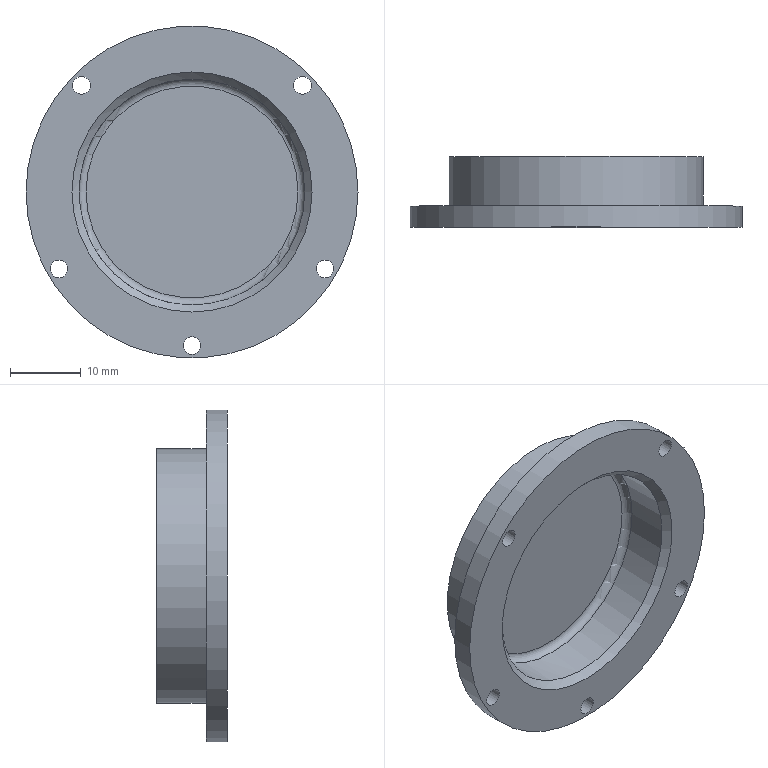Component | NX | FLANGE | 1 solid | 14 faces | box 47 x 10 x 47 mm | volume 5792 mm3 | cylinder 8 | plane 4 | cone 1 | torus 1 | commonest cylinder face diameters 2.5 x5 36 x1 47 x1 32 x1
STEP:
#1=CARTESIAN_POINT('',(0.,0.,0.));
#2=DIRECTION('',(0.,0.,1.));
#3=DIRECTION('',(1.,0.,0.));
#4=AXIS2_PLACEMENT_3D('',#1,#2,#3);
#5=CARTESIAN_POINT('',(-14.395,-16.2,58.409));
#6=VERTEX_POINT('',#5);
#7=CARTESIAN_POINT('',(-15.645,-16.2,58.409));
#8=DIRECTION('',(0.,1.,0.));
#9=DIRECTION('',(1.,0.,0.));
#10=AXIS2_PLACEMENT_3D('',#7,#8,#9);
#11=CIRCLE('',#10,1.25);
#12=CARTESIAN_POINT('',(0.0005589,-16.2,43.3));
#13=DIRECTION('',(0.,-1.,0.));
#14=DIRECTION('',(1.,0.,0.));
#15=AXIS2_PLACEMENT_3D('',#12,#13,#14);
#16=PLANE('',#15);
#17=CARTESIAN_POINT('',(-14.396,15.109));
#18=CARTESIAN_POINT('',(-14.396,12.944));
#19=CARTESIAN_POINT('',(-16.271,14.026));
#20=CARTESIAN_POINT('',(-18.146,15.109));
#21=CARTESIAN_POINT('',(-16.271,16.191));
#22=CARTESIAN_POINT('',(-14.396,17.274));
#23=CARTESIAN_POINT('',(-14.396,15.109));
#24=(BOUNDED_CURVE()B_SPLINE_CURVE(2,(#17,#18,#19,#20,#21,#22,#23),.UNSPECIFIED.,.T.,.F.)B_SPLINE_CURVE_WITH_KNOTS((1,2,2,2,2,1),(-2.094,0.,2.094,4.189,6.283,8.378),.UNSPECIFIED.)CURVE()GEOMETRIC_REPRESENTATION_ITEM()RATIONAL_B_SPLINE_CURVE((1.,0.5,1.,0.5,1.,0.5,1.))REPRESENTATION_ITEM(''));
#25=(GEOMETRIC_REPRESENTATION_CONTEXT(2)PARAMETRIC_REPRESENTATION_CONTEXT()REPRESENTATION_CONTEXT('',''));
#26=DEFINITIONAL_REPRESENTATION('',(#24),#25);
#27=PCURVE('',#16,#26);
#28=CARTESIAN_POINT('',(-15.645,-8.2,58.409));
#29=DIRECTION('',(0.,-1.,0.));
#30=DIRECTION('',(1.,0.,0.));
#31=AXIS2_PLACEMENT_3D('',#28,#29,#30);
#32=CYLINDRICAL_SURFACE('',#31,1.25);
#33=CARTESIAN_POINT('',(6.283,8.));
#34=DIRECTION('',(-1.,0.));
#35=VECTOR('',#34,1.);
#36=LINE('',#33,#35);
#37=(GEOMETRIC_REPRESENTATION_CONTEXT(2)PARAMETRIC_REPRESENTATION_CONTEXT()REPRESENTATION_CONTEXT('',''));
#38=DEFINITIONAL_REPRESENTATION('',(#36),#37);
#39=PCURVE('',#32,#38);
#40=SURFACE_CURVE('',#11,(#27,#39),.PCURVE_S1.);
#41=EDGE_CURVE('',#6,#6,#40,.T.);
#42=ORIENTED_EDGE('',*,*,#41,.T.);
#43=EDGE_LOOP('',(#42));
#44=FACE_BOUND('',#43,.T.);
#45=CARTESIAN_POINT('',(-17.585,-16.2,32.425));
#46=VERTEX_POINT('',#45);
#47=CARTESIAN_POINT('',(-18.835,-16.2,32.425));
#48=DIRECTION('',(0.,1.,0.));
#49=DIRECTION('',(1.,0.,0.));
#50=AXIS2_PLACEMENT_3D('',#47,#48,#49);
#51=CIRCLE('',#50,1.25);
#52=CARTESIAN_POINT('',(-17.586,-10.875));
#53=CARTESIAN_POINT('',(-17.586,-13.04));
#54=CARTESIAN_POINT('',(-19.461,-11.958));
#55=CARTESIAN_POINT('',(-21.336,-10.875));
#56=CARTESIAN_POINT('',(-19.461,-9.792));
#57=CARTESIAN_POINT('',(-17.586,-8.71));
#58=CARTESIAN_POINT('',(-17.586,-10.875));
#59=(BOUNDED_CURVE()B_SPLINE_CURVE(2,(#52,#53,#54,#55,#56,#57,#58),.UNSPECIFIED.,.T.,.F.)B_SPLINE_CURVE_WITH_KNOTS((1,2,2,2,2,1),(-2.094,0.,2.094,4.189,6.283,8.378),.UNSPECIFIED.)CURVE()GEOMETRIC_REPRESENTATION_ITEM()RATIONAL_B_SPLINE_CURVE((1.,0.5,1.,0.5,1.,0.5,1.))REPRESENTATION_ITEM(''));
#60=(GEOMETRIC_REPRESENTATION_CONTEXT(2)PARAMETRIC_REPRESENTATION_CONTEXT()REPRESENTATION_CONTEXT('',''));
#61=DEFINITIONAL_REPRESENTATION('',(#59),#60);
#62=PCURVE('',#16,#61);
#63=CARTESIAN_POINT('',(-18.835,-8.2,32.425));
#64=DIRECTION('',(0.,-1.,0.));
#65=DIRECTION('',(1.,0.,0.));
#66=AXIS2_PLACEMENT_3D('',#63,#64,#65);
#67=CYLINDRICAL_SURFACE('',#66,1.25);
#68=CARTESIAN_POINT('',(6.283,8.));
#69=DIRECTION('',(-1.,0.));
#70=VECTOR('',#69,1.);
#71=LINE('',#68,#70);
#72=(GEOMETRIC_REPRESENTATION_CONTEXT(2)PARAMETRIC_REPRESENTATION_CONTEXT()REPRESENTATION_CONTEXT('',''));
#73=DEFINITIONAL_REPRESENTATION('',(#71),#72);
#74=PCURVE('',#67,#73);
#75=SURFACE_CURVE('',#51,(#62,#74),.PCURVE_S1.);
#76=EDGE_CURVE('',#46,#46,#75,.T.);
#77=ORIENTED_EDGE('',*,*,#76,.T.);
#78=EDGE_LOOP('',(#77));
#79=FACE_BOUND('',#78,.T.);
#80=CARTESIAN_POINT('',(1.251,-16.2,21.55));
#81=VERTEX_POINT('',#80);
#82=CARTESIAN_POINT('',(0.0005589,-16.2,21.55));
#83=DIRECTION('',(0.,1.,0.));
#84=DIRECTION('',(1.,0.,0.));
#85=AXIS2_PLACEMENT_3D('',#82,#83,#84);
#86=CIRCLE('',#85,1.25);
#87=CARTESIAN_POINT('',(1.25,-21.75));
#88=CARTESIAN_POINT('',(1.25,-23.915));
#89=CARTESIAN_POINT('',(-0.625,-22.833));
#90=CARTESIAN_POINT('',(-2.5,-21.75));
#91=CARTESIAN_POINT('',(-0.625,-20.667));
#92=CARTESIAN_POINT('',(1.25,-19.585));
#93=CARTESIAN_POINT('',(1.25,-21.75));
#94=(BOUNDED_CURVE()B_SPLINE_CURVE(2,(#87,#88,#89,#90,#91,#92,#93),.UNSPECIFIED.,.T.,.F.)B_SPLINE_CURVE_WITH_KNOTS((1,2,2,2,2,1),(-2.094,0.,2.094,4.189,6.283,8.378),.UNSPECIFIED.)CURVE()GEOMETRIC_REPRESENTATION_ITEM()RATIONAL_B_SPLINE_CURVE((1.,0.5,1.,0.5,1.,0.5,1.))REPRESENTATION_ITEM(''));
#95=(GEOMETRIC_REPRESENTATION_CONTEXT(2)PARAMETRIC_REPRESENTATION_CONTEXT()REPRESENTATION_CONTEXT('',''));
#96=DEFINITIONAL_REPRESENTATION('',(#94),#95);
#97=PCURVE('',#16,#96);
#98=CARTESIAN_POINT('',(0.0005589,-8.2,21.55));
#99=DIRECTION('',(0.,-1.,0.));
#100=DIRECTION('',(1.,0.,0.));
#101=AXIS2_PLACEMENT_3D('',#98,#99,#100);
#102=CYLINDRICAL_SURFACE('',#101,1.25);
#103=CARTESIAN_POINT('',(6.283,8.));
#104=DIRECTION('',(-1.,0.));
#105=VECTOR('',#104,1.);
#106=LINE('',#103,#105);
#107=(GEOMETRIC_REPRESENTATION_CONTEXT(2)PARAMETRIC_REPRESENTATION_CONTEXT()REPRESENTATION_CONTEXT('',''));
#108=DEFINITIONAL_REPRESENTATION('',(#106),#107);
#109=PCURVE('',#102,#108);
#110=SURFACE_CURVE('',#86,(#97,#109),.PCURVE_S1.);
#111=EDGE_CURVE('',#81,#81,#110,.T.);
#112=ORIENTED_EDGE('',*,*,#111,.T.);
#113=EDGE_LOOP('',(#112));
#114=FACE_BOUND('',#113,.T.);
#115=CARTESIAN_POINT('',(17.001,-16.2,43.3));
#116=VERTEX_POINT('',#115);
#117=CARTESIAN_POINT('',(0.0005589,-16.2,43.3));
#118=DIRECTION('',(0.,1.,0.));
#119=DIRECTION('',(1.,0.,0.));
#120=AXIS2_PLACEMENT_3D('',#117,#118,#119);
#121=CIRCLE('',#120,17.);
#122=CARTESIAN_POINT('',(17.,0.));
#123=CARTESIAN_POINT('',(17.,-29.445));
#124=CARTESIAN_POINT('',(-8.5,-14.722));
#125=CARTESIAN_POINT('',(-34.,-0.));
#126=CARTESIAN_POINT('',(-8.5,14.722));
#127=CARTESIAN_POINT('',(17.,29.445));
#128=CARTESIAN_POINT('',(17.,0.));
#129=(BOUNDED_CURVE()B_SPLINE_CURVE(2,(#122,#123,#124,#125,#126,#127,#128),.UNSPECIFIED.,.T.,.F.)B_SPLINE_CURVE_WITH_KNOTS((1,2,2,2,2,1),(-2.094,0.,2.094,4.189,6.283,8.378),.UNSPECIFIED.)CURVE()GEOMETRIC_REPRESENTATION_ITEM()RATIONAL_B_SPLINE_CURVE((1.,0.5,1.,0.5,1.,0.5,1.))REPRESENTATION_ITEM(''));
#130=(GEOMETRIC_REPRESENTATION_CONTEXT(2)PARAMETRIC_REPRESENTATION_CONTEXT()REPRESENTATION_CONTEXT('',''));
#131=DEFINITIONAL_REPRESENTATION('',(#129),#130);
#132=PCURVE('',#16,#131);
#133=CARTESIAN_POINT('',(0.0005589,-16.2,43.3));
#134=DIRECTION('',(0.,-1.,0.));
#135=DIRECTION('',(1.,0.,0.));
#136=AXIS2_PLACEMENT_3D('',#133,#134,#135);
#137=CONICAL_SURFACE('',#136,17.,0.7854);
#138=CARTESIAN_POINT('',(6.283,0.));
#139=DIRECTION('',(-1.,0.));
#140=VECTOR('',#139,1.);
#141=LINE('',#138,#140);
#142=(GEOMETRIC_REPRESENTATION_CONTEXT(2)PARAMETRIC_REPRESENTATION_CONTEXT()REPRESENTATION_CONTEXT('',''));
#143=DEFINITIONAL_REPRESENTATION('',(#141),#142);
#144=PCURVE('',#137,#143);
#145=SURFACE_CURVE('',#121,(#132,#144),.PCURVE_S1.);
#146=EDGE_CURVE('',#116,#116,#145,.T.);
#147=ORIENTED_EDGE('',*,*,#146,.T.);
#148=EDGE_LOOP('',(#147));
#149=FACE_BOUND('',#148,.T.);
#150=CARTESIAN_POINT('',(23.501,-16.2,43.3));
#151=VERTEX_POINT('',#150);
#152=CARTESIAN_POINT('',(0.0005589,-16.2,43.3));
#153=DIRECTION('',(0.,-1.,0.));
#154=DIRECTION('',(1.,0.,0.));
#155=AXIS2_PLACEMENT_3D('',#152,#153,#154);
#156=CIRCLE('',#155,23.5);
#157=CARTESIAN_POINT('',(0.,0.));
#158=DIRECTION('',(1.,0.));
#159=AXIS2_PLACEMENT_2D('',#157,#158);
#160=CIRCLE('',#159,23.5);
#161=(GEOMETRIC_REPRESENTATION_CONTEXT(2)PARAMETRIC_REPRESENTATION_CONTEXT()REPRESENTATION_CONTEXT('',''));
#162=DEFINITIONAL_REPRESENTATION('',(#160),#161);
#163=PCURVE('',#16,#162);
#164=CARTESIAN_POINT('',(0.0005589,-13.2,43.3));
#165=DIRECTION('',(0.,-1.,0.));
#166=DIRECTION('',(1.,0.,0.));
#167=AXIS2_PLACEMENT_3D('',#164,#165,#166);
#168=CYLINDRICAL_SURFACE('',#167,23.5);
#169=CARTESIAN_POINT('',(0.,3.));
#170=DIRECTION('',(1.,0.));
#171=VECTOR('',#170,1.);
#172=LINE('',#169,#171);
#173=(GEOMETRIC_REPRESENTATION_CONTEXT(2)PARAMETRIC_REPRESENTATION_CONTEXT()REPRESENTATION_CONTEXT('',''));
#174=DEFINITIONAL_REPRESENTATION('',(#172),#173);
#175=PCURVE('',#168,#174);
#176=SURFACE_CURVE('',#156,(#163,#175),.PCURVE_S1.);
#177=EDGE_CURVE('',#151,#151,#176,.T.);
#178=ORIENTED_EDGE('',*,*,#177,.T.);
#179=EDGE_LOOP('',(#178));
#180=FACE_BOUND('',#179,.T.);
#181=CARTESIAN_POINT('',(14.396,-16.2,58.409));
#182=VERTEX_POINT('',#181);
#183=CARTESIAN_POINT('',(15.646,-16.2,58.409));
#184=DIRECTION('',(0.,-1.,0.));
#185=DIRECTION('',(-1.,0.,0.));
#186=AXIS2_PLACEMENT_3D('',#183,#184,#185);
#187=CIRCLE('',#186,1.25);
#188=CARTESIAN_POINT('',(15.646,15.109));
#189=DIRECTION('',(-1.,0.));
#190=AXIS2_PLACEMENT_2D('',#188,#189);
#191=CIRCLE('',#190,1.25);
#192=(GEOMETRIC_REPRESENTATION_CONTEXT(2)PARAMETRIC_REPRESENTATION_CONTEXT()REPRESENTATION_CONTEXT('',''));
#193=DEFINITIONAL_REPRESENTATION('',(#191),#192);
#194=PCURVE('',#16,#193);
#195=CARTESIAN_POINT('',(15.646,-8.2,58.409));
#196=DIRECTION('',(0.,-1.,0.));
#197=DIRECTION('',(1.,0.,0.));
#198=AXIS2_PLACEMENT_3D('',#195,#196,#197);
#199=CYLINDRICAL_SURFACE('',#198,1.25);
#200=CARTESIAN_POINT('',(3.142,8.));
#201=DIRECTION('',(1.,0.));
#202=VECTOR('',#201,1.);
#203=LINE('',#200,#202);
#204=(GEOMETRIC_REPRESENTATION_CONTEXT(2)PARAMETRIC_REPRESENTATION_CONTEXT()REPRESENTATION_CONTEXT('',''));
#205=DEFINITIONAL_REPRESENTATION('',(#203),#204);
#206=PCURVE('',#199,#205);
#207=SURFACE_CURVE('',#187,(#194,#206),.PCURVE_S1.);
#208=EDGE_CURVE('',#182,#182,#207,.T.);
#209=ORIENTED_EDGE('',*,*,#208,.F.);
#210=EDGE_LOOP('',(#209));
#211=FACE_BOUND('',#210,.T.);
#212=CARTESIAN_POINT('',(17.587,-16.2,32.425));
#213=VERTEX_POINT('',#212);
#214=CARTESIAN_POINT('',(18.837,-16.2,32.425));
#215=DIRECTION('',(0.,-1.,0.));
#216=DIRECTION('',(-1.,0.,0.));
#217=AXIS2_PLACEMENT_3D('',#214,#215,#216);
#218=CIRCLE('',#217,1.25);
#219=CARTESIAN_POINT('',(18.836,-10.875));
#220=DIRECTION('',(-1.,0.));
#221=AXIS2_PLACEMENT_2D('',#219,#220);
#222=CIRCLE('',#221,1.25);
#223=(GEOMETRIC_REPRESENTATION_CONTEXT(2)PARAMETRIC_REPRESENTATION_CONTEXT()REPRESENTATION_CONTEXT('',''));
#224=DEFINITIONAL_REPRESENTATION('',(#222),#223);
#225=PCURVE('',#16,#224);
#226=CARTESIAN_POINT('',(18.837,-8.2,32.425));
#227=DIRECTION('',(0.,-1.,0.));
#228=DIRECTION('',(1.,0.,0.));
#229=AXIS2_PLACEMENT_3D('',#226,#227,#228);
#230=CYLINDRICAL_SURFACE('',#229,1.25);
#231=CARTESIAN_POINT('',(3.142,8.));
#232=DIRECTION('',(1.,0.));
#233=VECTOR('',#232,1.);
#234=LINE('',#231,#233);
#235=(GEOMETRIC_REPRESENTATION_CONTEXT(2)PARAMETRIC_REPRESENTATION_CONTEXT()REPRESENTATION_CONTEXT('',''));
#236=DEFINITIONAL_REPRESENTATION('',(#234),#235);
#237=PCURVE('',#230,#236);
#238=SURFACE_CURVE('',#218,(#225,#237),.PCURVE_S1.);
#239=EDGE_CURVE('',#213,#213,#238,.T.);
#240=ORIENTED_EDGE('',*,*,#239,.F.);
#241=EDGE_LOOP('',(#240));
#242=FACE_BOUND('',#241,.T.);
#243=ADVANCED_FACE('',(#44,#79,#114,#149,#180,#211,#242),#16,.T.);
#244=CARTESIAN_POINT('',(-16.895,-13.2,58.409));
#245=VERTEX_POINT('',#244);
#246=CARTESIAN_POINT('',(-14.395,-13.2,58.409));
#247=VERTEX_POINT('',#246);
#248=CARTESIAN_POINT('',(-15.645,-13.2,58.409));
#249=DIRECTION('',(0.,-1.,0.));
#250=DIRECTION('',(-1.,0.,0.));
#251=AXIS2_PLACEMENT_3D('',#248,#249,#250);
#252=CIRCLE('',#251,1.25);
#253=CARTESIAN_POINT('',(0.0005589,-13.2,43.3));
#254=DIRECTION('',(0.,1.,0.));
#255=DIRECTION('',(-1.,0.,0.));
#256=AXIS2_PLACEMENT_3D('',#253,#254,#255);
#257=PLANE('',#256);
#258=CARTESIAN_POINT('',(16.896,15.109));
#259=CARTESIAN_POINT('',(16.896,12.944));
#260=CARTESIAN_POINT('',(15.021,14.026));
#261=CARTESIAN_POINT('',(13.146,15.109));
#262=CARTESIAN_POINT('',(15.021,16.191));
#263=CARTESIAN_POINT('',(16.896,17.274));
#264=CARTESIAN_POINT('',(16.896,15.109));
#265=(BOUNDED_CURVE()B_SPLINE_CURVE(2,(#258,#259,#260,#261,#262,#263,#264),.UNSPECIFIED.,.T.,.F.)B_SPLINE_CURVE_WITH_KNOTS((1,2,2,2,2,1),(-2.094,0.,2.094,4.189,6.283,8.378),.UNSPECIFIED.)CURVE()GEOMETRIC_REPRESENTATION_ITEM()RATIONAL_B_SPLINE_CURVE((1.,0.5,1.,0.5,1.,0.5,1.))REPRESENTATION_ITEM(''));
#266=(GEOMETRIC_REPRESENTATION_CONTEXT(2)PARAMETRIC_REPRESENTATION_CONTEXT()REPRESENTATION_CONTEXT('',''));
#267=DEFINITIONAL_REPRESENTATION('',(#265),#266);
#268=PCURVE('',#257,#267);
#269=CARTESIAN_POINT('',(3.142,5.));
#270=DIRECTION('',(1.,0.));
#271=VECTOR('',#270,1.);
#272=LINE('',#269,#271);
#273=(GEOMETRIC_REPRESENTATION_CONTEXT(2)PARAMETRIC_REPRESENTATION_CONTEXT()REPRESENTATION_CONTEXT('',''));
#274=DEFINITIONAL_REPRESENTATION('',(#272),#273);
#275=PCURVE('',#32,#274);
#276=SURFACE_CURVE('',#252,(#268,#275),.PCURVE_S1.);
#277=EDGE_CURVE('',#245,#247,#276,.T.);
#278=ORIENTED_EDGE('',*,*,#277,.T.);
#279=CARTESIAN_POINT('',(-15.645,-13.2,58.409));
#280=DIRECTION('',(0.,-1.,0.));
#281=DIRECTION('',(-1.,0.,0.));
#282=AXIS2_PLACEMENT_3D('',#279,#280,#281);
#283=CIRCLE('',#282,1.25);
#284=CARTESIAN_POINT('',(16.896,15.109));
#285=CARTESIAN_POINT('',(16.896,12.944));
#286=CARTESIAN_POINT('',(15.021,14.026));
#287=CARTESIAN_POINT('',(13.146,15.109));
#288=CARTESIAN_POINT('',(15.021,16.191));
#289=CARTESIAN_POINT('',(16.896,17.274));
#290=CARTESIAN_POINT('',(16.896,15.109));
#291=(BOUNDED_CURVE()B_SPLINE_CURVE(2,(#284,#285,#286,#287,#288,#289,#290),.UNSPECIFIED.,.T.,.F.)B_SPLINE_CURVE_WITH_KNOTS((1,2,2,2,2,1),(-2.094,0.,2.094,4.189,6.283,8.378),.UNSPECIFIED.)CURVE()GEOMETRIC_REPRESENTATION_ITEM()RATIONAL_B_SPLINE_CURVE((1.,0.5,1.,0.5,1.,0.5,1.))REPRESENTATION_ITEM(''));
#292=(GEOMETRIC_REPRESENTATION_CONTEXT(2)PARAMETRIC_REPRESENTATION_CONTEXT()REPRESENTATION_CONTEXT('',''));
#293=DEFINITIONAL_REPRESENTATION('',(#291),#292);
#294=PCURVE('',#257,#293);
#295=CARTESIAN_POINT('',(-3.142,5.));
#296=DIRECTION('',(1.,0.));
#297=VECTOR('',#296,1.);
#298=LINE('',#295,#297);
#299=(GEOMETRIC_REPRESENTATION_CONTEXT(2)PARAMETRIC_REPRESENTATION_CONTEXT()REPRESENTATION_CONTEXT('',''));
#300=DEFINITIONAL_REPRESENTATION('',(#298),#299);
#301=PCURVE('',#32,#300);
#302=SURFACE_CURVE('',#283,(#294,#301),.PCURVE_S1.);
#303=EDGE_CURVE('',#247,#245,#302,.T.);
#304=ORIENTED_EDGE('',*,*,#303,.T.);
#305=EDGE_LOOP('',(#278,#304));
#306=FACE_BOUND('',#305,.T.);
#307=CARTESIAN_POINT('',(-20.085,-13.2,32.425));
#308=VERTEX_POINT('',#307);
#309=CARTESIAN_POINT('',(-17.585,-13.2,32.425));
#310=VERTEX_POINT('',#309);
#311=CARTESIAN_POINT('',(-18.835,-13.2,32.425));
#312=DIRECTION('',(0.,-1.,0.));
#313=DIRECTION('',(-1.,0.,0.));
#314=AXIS2_PLACEMENT_3D('',#311,#312,#313);
#315=CIRCLE('',#314,1.25);
#316=CARTESIAN_POINT('',(20.086,-10.875));
#317=CARTESIAN_POINT('',(20.086,-13.04));
#318=CARTESIAN_POINT('',(18.211,-11.958));
#319=CARTESIAN_POINT('',(16.336,-10.875));
#320=CARTESIAN_POINT('',(18.211,-9.792));
#321=CARTESIAN_POINT('',(20.086,-8.71));
#322=CARTESIAN_POINT('',(20.086,-10.875));
#323=(BOUNDED_CURVE()B_SPLINE_CURVE(2,(#316,#317,#318,#319,#320,#321,#322),.UNSPECIFIED.,.T.,.F.)B_SPLINE_CURVE_WITH_KNOTS((1,2,2,2,2,1),(-2.094,0.,2.094,4.189,6.283,8.378),.UNSPECIFIED.)CURVE()GEOMETRIC_REPRESENTATION_ITEM()RATIONAL_B_SPLINE_CURVE((1.,0.5,1.,0.5,1.,0.5,1.))REPRESENTATION_ITEM(''));
#324=(GEOMETRIC_REPRESENTATION_CONTEXT(2)PARAMETRIC_REPRESENTATION_CONTEXT()REPRESENTATION_CONTEXT('',''));
#325=DEFINITIONAL_REPRESENTATION('',(#323),#324);
#326=PCURVE('',#257,#325);
#327=CARTESIAN_POINT('',(3.142,5.));
#328=DIRECTION('',(1.,0.));
#329=VECTOR('',#328,1.);
#330=LINE('',#327,#329);
#331=(GEOMETRIC_REPRESENTATION_CONTEXT(2)PARAMETRIC_REPRESENTATION_CONTEXT()REPRESENTATION_CONTEXT('',''));
#332=DEFINITIONAL_REPRESENTATION('',(#330),#331);
#333=PCURVE('',#67,#332);
#334=SURFACE_CURVE('',#315,(#326,#333),.PCURVE_S1.);
#335=EDGE_CURVE('',#308,#310,#334,.T.);
#336=ORIENTED_EDGE('',*,*,#335,.T.);
#337=CARTESIAN_POINT('',(-18.835,-13.2,32.425));
#338=DIRECTION('',(0.,-1.,0.));
#339=DIRECTION('',(-1.,0.,0.));
#340=AXIS2_PLACEMENT_3D('',#337,#338,#339);
#341=CIRCLE('',#340,1.25);
#342=CARTESIAN_POINT('',(20.086,-10.875));
#343=CARTESIAN_POINT('',(20.086,-13.04));
#344=CARTESIAN_POINT('',(18.211,-11.958));
#345=CARTESIAN_POINT('',(16.336,-10.875));
#346=CARTESIAN_POINT('',(18.211,-9.792));
#347=CARTESIAN_POINT('',(20.086,-8.71));
#348=CARTESIAN_POINT('',(20.086,-10.875));
#349=(BOUNDED_CURVE()B_SPLINE_CURVE(2,(#342,#343,#344,#345,#346,#347,#348),.UNSPECIFIED.,.T.,.F.)B_SPLINE_CURVE_WITH_KNOTS((1,2,2,2,2,1),(-2.094,0.,2.094,4.189,6.283,8.378),.UNSPECIFIED.)CURVE()GEOMETRIC_REPRESENTATION_ITEM()RATIONAL_B_SPLINE_CURVE((1.,0.5,1.,0.5,1.,0.5,1.))REPRESENTATION_ITEM(''));
#350=(GEOMETRIC_REPRESENTATION_CONTEXT(2)PARAMETRIC_REPRESENTATION_CONTEXT()REPRESENTATION_CONTEXT('',''));
#351=DEFINITIONAL_REPRESENTATION('',(#349),#350);
#352=PCURVE('',#257,#351);
#353=CARTESIAN_POINT('',(-3.142,5.));
#354=DIRECTION('',(1.,0.));
#355=VECTOR('',#354,1.);
#356=LINE('',#353,#355);
#357=(GEOMETRIC_REPRESENTATION_CONTEXT(2)PARAMETRIC_REPRESENTATION_CONTEXT()REPRESENTATION_CONTEXT('',''));
#358=DEFINITIONAL_REPRESENTATION('',(#356),#357);
#359=PCURVE('',#67,#358);
#360=SURFACE_CURVE('',#341,(#352,#359),.PCURVE_S1.);
#361=EDGE_CURVE('',#310,#308,#360,.T.);
#362=ORIENTED_EDGE('',*,*,#361,.T.);
#363=EDGE_LOOP('',(#336,#362));
#364=FACE_BOUND('',#363,.T.);
#365=CARTESIAN_POINT('',(-1.249,-13.2,21.55));
#366=VERTEX_POINT('',#365);
#367=CARTESIAN_POINT('',(1.251,-13.2,21.55));
#368=VERTEX_POINT('',#367);
#369=CARTESIAN_POINT('',(0.0005589,-13.2,21.55));
#370=DIRECTION('',(0.,-1.,0.));
#371=DIRECTION('',(-1.,0.,0.));
#372=AXIS2_PLACEMENT_3D('',#369,#370,#371);
#373=CIRCLE('',#372,1.25);
#374=CARTESIAN_POINT('',(1.25,-21.75));
#375=CARTESIAN_POINT('',(1.25,-23.915));
#376=CARTESIAN_POINT('',(-0.625,-22.833));
#377=CARTESIAN_POINT('',(-2.5,-21.75));
#378=CARTESIAN_POINT('',(-0.625,-20.667));
#379=CARTESIAN_POINT('',(1.25,-19.585));
#380=CARTESIAN_POINT('',(1.25,-21.75));
#381=(BOUNDED_CURVE()B_SPLINE_CURVE(2,(#374,#375,#376,#377,#378,#379,#380),.UNSPECIFIED.,.T.,.F.)B_SPLINE_CURVE_WITH_KNOTS((1,2,2,2,2,1),(-2.094,0.,2.094,4.189,6.283,8.378),.UNSPECIFIED.)CURVE()GEOMETRIC_REPRESENTATION_ITEM()RATIONAL_B_SPLINE_CURVE((1.,0.5,1.,0.5,1.,0.5,1.))REPRESENTATION_ITEM(''));
#382=(GEOMETRIC_REPRESENTATION_CONTEXT(2)PARAMETRIC_REPRESENTATION_CONTEXT()REPRESENTATION_CONTEXT('',''));
#383=DEFINITIONAL_REPRESENTATION('',(#381),#382);
#384=PCURVE('',#257,#383);
#385=CARTESIAN_POINT('',(3.142,5.));
#386=DIRECTION('',(1.,0.));
#387=VECTOR('',#386,1.);
#388=LINE('',#385,#387);
#389=(GEOMETRIC_REPRESENTATION_CONTEXT(2)PARAMETRIC_REPRESENTATION_CONTEXT()REPRESENTATION_CONTEXT('',''));
#390=DEFINITIONAL_REPRESENTATION('',(#388),#389);
#391=PCURVE('',#102,#390);
#392=SURFACE_CURVE('',#373,(#384,#391),.PCURVE_S1.);
#393=EDGE_CURVE('',#366,#368,#392,.T.);
#394=ORIENTED_EDGE('',*,*,#393,.T.);
#395=CARTESIAN_POINT('',(0.0005589,-13.2,21.55));
#396=DIRECTION('',(0.,-1.,0.));
#397=DIRECTION('',(-1.,0.,0.));
#398=AXIS2_PLACEMENT_3D('',#395,#396,#397);
#399=CIRCLE('',#398,1.25);
#400=CARTESIAN_POINT('',(1.25,-21.75));
#401=CARTESIAN_POINT('',(1.25,-23.915));
#402=CARTESIAN_POINT('',(-0.625,-22.833));
#403=CARTESIAN_POINT('',(-2.5,-21.75));
#404=CARTESIAN_POINT('',(-0.625,-20.667));
#405=CARTESIAN_POINT('',(1.25,-19.585));
#406=CARTESIAN_POINT('',(1.25,-21.75));
#407=(BOUNDED_CURVE()B_SPLINE_CURVE(2,(#400,#401,#402,#403,#404,#405,#406),.UNSPECIFIED.,.T.,.F.)B_SPLINE_CURVE_WITH_KNOTS((1,2,2,2,2,1),(-2.094,0.,2.094,4.189,6.283,8.378),.UNSPECIFIED.)CURVE()GEOMETRIC_REPRESENTATION_ITEM()RATIONAL_B_SPLINE_CURVE((1.,0.5,1.,0.5,1.,0.5,1.))REPRESENTATION_ITEM(''));
#408=(GEOMETRIC_REPRESENTATION_CONTEXT(2)PARAMETRIC_REPRESENTATION_CONTEXT()REPRESENTATION_CONTEXT('',''));
#409=DEFINITIONAL_REPRESENTATION('',(#407),#408);
#410=PCURVE('',#257,#409);
#411=CARTESIAN_POINT('',(-3.142,5.));
#412=DIRECTION('',(1.,0.));
#413=VECTOR('',#412,1.);
#414=LINE('',#411,#413);
#415=(GEOMETRIC_REPRESENTATION_CONTEXT(2)PARAMETRIC_REPRESENTATION_CONTEXT()REPRESENTATION_CONTEXT('',''));
#416=DEFINITIONAL_REPRESENTATION('',(#414),#415);
#417=PCURVE('',#102,#416);
#418=SURFACE_CURVE('',#399,(#410,#417),.PCURVE_S1.);
#419=EDGE_CURVE('',#368,#366,#418,.T.);
#420=ORIENTED_EDGE('',*,*,#419,.T.);
#421=EDGE_LOOP('',(#394,#420));
#422=FACE_BOUND('',#421,.T.);
#423=CARTESIAN_POINT('',(18.001,-13.2,43.3));
#424=VERTEX_POINT('',#423);
#425=CARTESIAN_POINT('',(0.0005589,-13.2,43.3));
#426=DIRECTION('',(0.,1.,0.));
#427=DIRECTION('',(1.,0.,0.));
#428=AXIS2_PLACEMENT_3D('',#425,#426,#427);
#429=CIRCLE('',#428,18.);
#430=CARTESIAN_POINT('',(0.,0.));
#431=DIRECTION('',(-1.,0.));
#432=AXIS2_PLACEMENT_2D('',#430,#431);
#433=CIRCLE('',#432,18.);
#434=(GEOMETRIC_REPRESENTATION_CONTEXT(2)PARAMETRIC_REPRESENTATION_CONTEXT()REPRESENTATION_CONTEXT('',''));
#435=DEFINITIONAL_REPRESENTATION('',(#433),#434);
#436=PCURVE('',#257,#435);
#437=CARTESIAN_POINT('',(0.0005589,-6.2,43.3));
#438=DIRECTION('',(0.,-1.,0.));
#439=DIRECTION('',(1.,0.,0.));
#440=AXIS2_PLACEMENT_3D('',#437,#438,#439);
#441=CYLINDRICAL_SURFACE('',#440,18.);
#442=CARTESIAN_POINT('',(6.283,7.));
#443=DIRECTION('',(-1.,0.));
#444=VECTOR('',#443,1.);
#445=LINE('',#442,#444);
#446=(GEOMETRIC_REPRESENTATION_CONTEXT(2)PARAMETRIC_REPRESENTATION_CONTEXT()REPRESENTATION_CONTEXT('',''));
#447=DEFINITIONAL_REPRESENTATION('',(#445),#446);
#448=PCURVE('',#441,#447);
#449=SURFACE_CURVE('',#429,(#436,#448),.PCURVE_S1.);
#450=EDGE_CURVE('',#424,#424,#449,.T.);
#451=ORIENTED_EDGE('',*,*,#450,.F.);
#452=EDGE_LOOP('',(#451));
#453=FACE_BOUND('',#452,.T.);
#454=CARTESIAN_POINT('',(23.501,-13.2,43.3));
#455=VERTEX_POINT('',#454);
#456=CARTESIAN_POINT('',(0.0005589,-13.2,43.3));
#457=DIRECTION('',(0.,-1.,0.));
#458=DIRECTION('',(1.,0.,0.));
#459=AXIS2_PLACEMENT_3D('',#456,#457,#458);
#460=CIRCLE('',#459,23.5);
#461=CARTESIAN_POINT('',(-23.5,0.));
#462=CARTESIAN_POINT('',(-23.5,40.703));
#463=CARTESIAN_POINT('',(11.75,20.352));
#464=CARTESIAN_POINT('',(47.,0.));
#465=CARTESIAN_POINT('',(11.75,-20.352));
#466=CARTESIAN_POINT('',(-23.5,-40.703));
#467=CARTESIAN_POINT('',(-23.5,0.));
#468=(BOUNDED_CURVE()B_SPLINE_CURVE(2,(#461,#462,#463,#464,#465,#466,#467),.UNSPECIFIED.,.T.,.F.)B_SPLINE_CURVE_WITH_KNOTS((1,2,2,2,2,1),(-2.094,0.,2.094,4.189,6.283,8.378),.UNSPECIFIED.)CURVE()GEOMETRIC_REPRESENTATION_ITEM()RATIONAL_B_SPLINE_CURVE((1.,0.5,1.,0.5,1.,0.5,1.))REPRESENTATION_ITEM(''));
#469=(GEOMETRIC_REPRESENTATION_CONTEXT(2)PARAMETRIC_REPRESENTATION_CONTEXT()REPRESENTATION_CONTEXT('',''));
#470=DEFINITIONAL_REPRESENTATION('',(#468),#469);
#471=PCURVE('',#257,#470);
#472=CARTESIAN_POINT('',(0.,0.));
#473=DIRECTION('',(1.,0.));
#474=VECTOR('',#473,1.);
#475=LINE('',#472,#474);
#476=(GEOMETRIC_REPRESENTATION_CONTEXT(2)PARAMETRIC_REPRESENTATION_CONTEXT()REPRESENTATION_CONTEXT('',''));
#477=DEFINITIONAL_REPRESENTATION('',(#475),#476);
#478=PCURVE('',#168,#477);
#479=SURFACE_CURVE('',#460,(#471,#478),.PCURVE_S1.);
#480=EDGE_CURVE('',#455,#455,#479,.T.);
#481=ORIENTED_EDGE('',*,*,#480,.F.);
#482=EDGE_LOOP('',(#481));
#483=FACE_BOUND('',#482,.T.);
#484=CARTESIAN_POINT('',(14.396,-13.2,58.409));
#485=VERTEX_POINT('',#484);
#486=CARTESIAN_POINT('',(15.646,-13.2,58.409));
#487=DIRECTION('',(0.,1.,0.));
#488=DIRECTION('',(-1.,0.,0.));
#489=AXIS2_PLACEMENT_3D('',#486,#487,#488);
#490=CIRCLE('',#489,1.25);
#491=CARTESIAN_POINT('',(-15.646,15.109));
#492=DIRECTION('',(1.,0.));
#493=AXIS2_PLACEMENT_2D('',#491,#492);
#494=CIRCLE('',#493,1.25);
#495=(GEOMETRIC_REPRESENTATION_CONTEXT(2)PARAMETRIC_REPRESENTATION_CONTEXT()REPRESENTATION_CONTEXT('',''));
#496=DEFINITIONAL_REPRESENTATION('',(#494),#495);
#497=PCURVE('',#257,#496);
#498=CARTESIAN_POINT('',(9.425,5.));
#499=DIRECTION('',(-1.,0.));
#500=VECTOR('',#499,1.);
#501=LINE('',#498,#500);
#502=(GEOMETRIC_REPRESENTATION_CONTEXT(2)PARAMETRIC_REPRESENTATION_CONTEXT()REPRESENTATION_CONTEXT('',''));
#503=DEFINITIONAL_REPRESENTATION('',(#501),#502);
#504=PCURVE('',#199,#503);
#505=SURFACE_CURVE('',#490,(#497,#504),.PCURVE_S1.);
#506=EDGE_CURVE('',#485,#485,#505,.T.);
#507=ORIENTED_EDGE('',*,*,#506,.F.);
#508=EDGE_LOOP('',(#507));
#509=FACE_BOUND('',#508,.T.);
#510=CARTESIAN_POINT('',(17.587,-13.2,32.425));
#511=VERTEX_POINT('',#510);
#512=CARTESIAN_POINT('',(18.837,-13.2,32.425));
#513=DIRECTION('',(0.,1.,0.));
#514=DIRECTION('',(-1.,0.,0.));
#515=AXIS2_PLACEMENT_3D('',#512,#513,#514);
#516=CIRCLE('',#515,1.25);
#517=CARTESIAN_POINT('',(-18.836,-10.875));
#518=DIRECTION('',(1.,0.));
#519=AXIS2_PLACEMENT_2D('',#517,#518);
#520=CIRCLE('',#519,1.25);
#521=(GEOMETRIC_REPRESENTATION_CONTEXT(2)PARAMETRIC_REPRESENTATION_CONTEXT()REPRESENTATION_CONTEXT('',''));
#522=DEFINITIONAL_REPRESENTATION('',(#520),#521);
#523=PCURVE('',#257,#522);
#524=CARTESIAN_POINT('',(9.425,5.));
#525=DIRECTION('',(-1.,0.));
#526=VECTOR('',#525,1.);
#527=LINE('',#524,#526);
#528=(GEOMETRIC_REPRESENTATION_CONTEXT(2)PARAMETRIC_REPRESENTATION_CONTEXT()REPRESENTATION_CONTEXT('',''));
#529=DEFINITIONAL_REPRESENTATION('',(#527),#528);
#530=PCURVE('',#230,#529);
#531=SURFACE_CURVE('',#516,(#523,#530),.PCURVE_S1.);
#532=EDGE_CURVE('',#511,#511,#531,.T.);
#533=ORIENTED_EDGE('',*,*,#532,.F.);
#534=EDGE_LOOP('',(#533));
#535=FACE_BOUND('',#534,.T.);
#536=ADVANCED_FACE('',(#306,#364,#422,#453,#483,#509,#535),#257,.T.);
#537=CARTESIAN_POINT('',(18.001,-6.2,43.3));
#538=VERTEX_POINT('',#537);
#539=CARTESIAN_POINT('',(0.0005589,-6.2,43.3));
#540=DIRECTION('',(0.,-1.,0.));
#541=DIRECTION('',(1.,0.,0.));
#542=AXIS2_PLACEMENT_3D('',#539,#540,#541);
#543=CIRCLE('',#542,18.);
#544=CARTESIAN_POINT('',(0.0005589,-6.2,43.3));
#545=DIRECTION('',(0.,1.,0.));
#546=DIRECTION('',(-1.,0.,0.));
#547=AXIS2_PLACEMENT_3D('',#544,#545,#546);
#548=PLANE('',#547);
#549=CARTESIAN_POINT('',(-18.,0.));
#550=CARTESIAN_POINT('',(-18.,31.177));
#551=CARTESIAN_POINT('',(9.,15.588));
#552=CARTESIAN_POINT('',(36.,0.));
#553=CARTESIAN_POINT('',(9.,-15.588));
#554=CARTESIAN_POINT('',(-18.,-31.177));
#555=CARTESIAN_POINT('',(-18.,0.));
#556=(BOUNDED_CURVE()B_SPLINE_CURVE(2,(#549,#550,#551,#552,#553,#554,#555),.UNSPECIFIED.,.T.,.F.)B_SPLINE_CURVE_WITH_KNOTS((1,2,2,2,2,1),(-2.094,0.,2.094,4.189,6.283,8.378),.UNSPECIFIED.)CURVE()GEOMETRIC_REPRESENTATION_ITEM()RATIONAL_B_SPLINE_CURVE((1.,0.5,1.,0.5,1.,0.5,1.))REPRESENTATION_ITEM(''));
#557=(GEOMETRIC_REPRESENTATION_CONTEXT(2)PARAMETRIC_REPRESENTATION_CONTEXT()REPRESENTATION_CONTEXT('',''));
#558=DEFINITIONAL_REPRESENTATION('',(#556),#557);
#559=PCURVE('',#548,#558);
#560=CARTESIAN_POINT('',(0.,0.));
#561=DIRECTION('',(1.,0.));
#562=VECTOR('',#561,1.);
#563=LINE('',#560,#562);
#564=(GEOMETRIC_REPRESENTATION_CONTEXT(2)PARAMETRIC_REPRESENTATION_CONTEXT()REPRESENTATION_CONTEXT('',''));
#565=DEFINITIONAL_REPRESENTATION('',(#563),#564);
#566=PCURVE('',#441,#565);
#567=SURFACE_CURVE('',#543,(#559,#566),.PCURVE_S1.);
#568=EDGE_CURVE('',#538,#538,#567,.T.);
#569=ORIENTED_EDGE('',*,*,#568,.F.);
#570=EDGE_LOOP('',(#569));
#571=FACE_BOUND('',#570,.T.);
#572=ADVANCED_FACE('',(#571),#548,.T.);
#573=ORIENTED_EDGE('',*,*,#450,.T.);
#574=CARTESIAN_POINT('',(18.001,-6.2,43.3));
#575=CARTESIAN_POINT('',(18.001,-13.2,43.3));
#576=B_SPLINE_CURVE_WITH_KNOTS('',1,(#574,#575),.UNSPECIFIED.,.F.,.F.,(2,2),(0.,7.),.PIECEWISE_BEZIER_KNOTS.);
#577=CARTESIAN_POINT('',(0.,0.));
#578=DIRECTION('',(0.,1.));
#579=VECTOR('',#578,1.);
#580=LINE('',#577,#579);
#581=(GEOMETRIC_REPRESENTATION_CONTEXT(2)PARAMETRIC_REPRESENTATION_CONTEXT()REPRESENTATION_CONTEXT('',''));
#582=DEFINITIONAL_REPRESENTATION('',(#580),#581);
#583=PCURVE('',#441,#582);
#584=CARTESIAN_POINT('',(6.283,0.));
#585=DIRECTION('',(0.,1.));
#586=VECTOR('',#585,1.);
#587=LINE('',#584,#586);
#588=(GEOMETRIC_REPRESENTATION_CONTEXT(2)PARAMETRIC_REPRESENTATION_CONTEXT()REPRESENTATION_CONTEXT('',''));
#589=DEFINITIONAL_REPRESENTATION('',(#587),#588);
#590=PCURVE('',#441,#589);
#591=SEAM_CURVE('',#576,(#583,#590),.PCURVE_S1.);
#592=EDGE_CURVE('',#538,#424,#591,.T.);
#593=ORIENTED_EDGE('',*,*,#592,.F.);
#594=ORIENTED_EDGE('',*,*,#568,.T.);
#595=ORIENTED_EDGE('',*,*,#592,.T.);
#596=EDGE_LOOP('',(#573,#593,#594,#595));
#597=FACE_BOUND('',#596,.T.);
#598=ADVANCED_FACE('',(#597),#441,.T.);
#599=ORIENTED_EDGE('',*,*,#177,.F.);
#600=CARTESIAN_POINT('',(23.501,-13.2,43.3));
#601=CARTESIAN_POINT('',(23.501,-16.2,43.3));
#602=B_SPLINE_CURVE_WITH_KNOTS('',1,(#600,#601),.UNSPECIFIED.,.F.,.F.,(2,2),(0.,3.),.PIECEWISE_BEZIER_KNOTS.);
#603=CARTESIAN_POINT('',(0.,0.));
#604=DIRECTION('',(0.,1.));
#605=VECTOR('',#604,1.);
#606=LINE('',#603,#605);
#607=(GEOMETRIC_REPRESENTATION_CONTEXT(2)PARAMETRIC_REPRESENTATION_CONTEXT()REPRESENTATION_CONTEXT('',''));
#608=DEFINITIONAL_REPRESENTATION('',(#606),#607);
#609=PCURVE('',#168,#608);
#610=CARTESIAN_POINT('',(6.283,0.));
#611=DIRECTION('',(0.,1.));
#612=VECTOR('',#611,1.);
#613=LINE('',#610,#612);
#614=(GEOMETRIC_REPRESENTATION_CONTEXT(2)PARAMETRIC_REPRESENTATION_CONTEXT()REPRESENTATION_CONTEXT('',''));
#615=DEFINITIONAL_REPRESENTATION('',(#613),#614);
#616=PCURVE('',#168,#615);
#617=SEAM_CURVE('',#602,(#609,#616),.PCURVE_S1.);
#618=EDGE_CURVE('',#455,#151,#617,.T.);
#619=ORIENTED_EDGE('',*,*,#618,.F.);
#620=ORIENTED_EDGE('',*,*,#480,.T.);
#621=ORIENTED_EDGE('',*,*,#618,.T.);
#622=EDGE_LOOP('',(#599,#619,#620,#621));
#623=FACE_BOUND('',#622,.T.);
#624=ADVANCED_FACE('',(#623),#168,.T.);
#625=CARTESIAN_POINT('',(16.001,-9.2,43.3));
#626=VERTEX_POINT('',#625);
#627=CARTESIAN_POINT('',(-15.999,-9.2,43.3));
#628=VERTEX_POINT('',#627);
#629=CARTESIAN_POINT('',(0.0005589,-9.2,43.3));
#630=DIRECTION('',(0.,1.,0.));
#631=DIRECTION('',(-1.,0.,0.));
#632=AXIS2_PLACEMENT_3D('',#629,#630,#631);
#633=CIRCLE('',#632,16.);
#634=CARTESIAN_POINT('',(0.0005589,-8.2,43.3));
#635=DIRECTION('',(0.,-1.,0.));
#636=DIRECTION('',(1.,0.,0.));
#637=AXIS2_PLACEMENT_3D('',#634,#635,#636);
#638=CYLINDRICAL_SURFACE('',#637,16.);
#639=CARTESIAN_POINT('',(9.425,1.));
#640=DIRECTION('',(-1.,0.));
#641=VECTOR('',#640,1.);
#642=LINE('',#639,#641);
#643=(GEOMETRIC_REPRESENTATION_CONTEXT(2)PARAMETRIC_REPRESENTATION_CONTEXT()REPRESENTATION_CONTEXT('',''));
#644=DEFINITIONAL_REPRESENTATION('',(#642),#643);
#645=PCURVE('',#638,#644);
#646=CARTESIAN_POINT('',(0.0005589,-9.2,43.3));
#647=DIRECTION('',(0.,1.,0.));
#648=DIRECTION('',(-1.,0.,0.));
#649=AXIS2_PLACEMENT_3D('',#646,#647,#648);
#650=TOROIDAL_SURFACE('',#649,15.,1.);
#651=CARTESIAN_POINT('',(0.,6.283));
#652=DIRECTION('',(1.,0.));
#653=VECTOR('',#652,1.);
#654=LINE('',#651,#653);
#655=(GEOMETRIC_REPRESENTATION_CONTEXT(2)PARAMETRIC_REPRESENTATION_CONTEXT()REPRESENTATION_CONTEXT('',''));
#656=DEFINITIONAL_REPRESENTATION('',(#654),#655);
#657=PCURVE('',#650,#656);
#658=SURFACE_CURVE('',#633,(#645,#657),.PCURVE_S1.);
#659=EDGE_CURVE('',#626,#628,#658,.T.);
#660=ORIENTED_EDGE('',*,*,#659,.F.);
#661=CARTESIAN_POINT('',(16.001,-15.2,43.3));
#662=VERTEX_POINT('',#661);
#663=CARTESIAN_POINT('',(16.001,-9.2,43.3));
#664=CARTESIAN_POINT('',(16.001,-15.2,43.3));
#665=B_SPLINE_CURVE_WITH_KNOTS('',1,(#663,#664),.UNSPECIFIED.,.F.,.F.,(2,2),(1.,7.),.PIECEWISE_BEZIER_KNOTS.);
#666=CARTESIAN_POINT('',(6.283,0.));
#667=DIRECTION('',(0.,1.));
#668=VECTOR('',#667,1.);
#669=LINE('',#666,#668);
#670=(GEOMETRIC_REPRESENTATION_CONTEXT(2)PARAMETRIC_REPRESENTATION_CONTEXT()REPRESENTATION_CONTEXT('',''));
#671=DEFINITIONAL_REPRESENTATION('',(#669),#670);
#672=PCURVE('',#638,#671);
#673=CARTESIAN_POINT('',(0.,0.));
#674=DIRECTION('',(0.,1.));
#675=VECTOR('',#674,1.);
#676=LINE('',#673,#675);
#677=(GEOMETRIC_REPRESENTATION_CONTEXT(2)PARAMETRIC_REPRESENTATION_CONTEXT()REPRESENTATION_CONTEXT('',''));
#678=DEFINITIONAL_REPRESENTATION('',(#676),#677);
#679=PCURVE('',#638,#678);
#680=SEAM_CURVE('',#665,(#672,#679),.PCURVE_S1.);
#681=EDGE_CURVE('',#626,#662,#680,.T.);
#682=ORIENTED_EDGE('',*,*,#681,.T.);
#683=CARTESIAN_POINT('',(0.0005589,-15.2,43.3));
#684=DIRECTION('',(0.,-1.,0.));
#685=DIRECTION('',(1.,0.,0.));
#686=AXIS2_PLACEMENT_3D('',#683,#684,#685);
#687=CIRCLE('',#686,16.);
#688=CARTESIAN_POINT('',(0.,7.));
#689=DIRECTION('',(1.,0.));
#690=VECTOR('',#689,1.);
#691=LINE('',#688,#690);
#692=(GEOMETRIC_REPRESENTATION_CONTEXT(2)PARAMETRIC_REPRESENTATION_CONTEXT()REPRESENTATION_CONTEXT('',''));
#693=DEFINITIONAL_REPRESENTATION('',(#691),#692);
#694=PCURVE('',#638,#693);
#695=CARTESIAN_POINT('',(0.,-1.));
#696=DIRECTION('',(1.,0.));
#697=VECTOR('',#696,1.);
#698=LINE('',#695,#697);
#699=(GEOMETRIC_REPRESENTATION_CONTEXT(2)PARAMETRIC_REPRESENTATION_CONTEXT()REPRESENTATION_CONTEXT('',''));
#700=DEFINITIONAL_REPRESENTATION('',(#698),#699);
#701=PCURVE('',#137,#700);
#702=SURFACE_CURVE('',#687,(#694,#701),.PCURVE_S1.);
#703=EDGE_CURVE('',#662,#662,#702,.T.);
#704=ORIENTED_EDGE('',*,*,#703,.F.);
#705=ORIENTED_EDGE('',*,*,#681,.F.);
#706=CARTESIAN_POINT('',(0.0005589,-9.2,43.3));
#707=DIRECTION('',(0.,1.,0.));
#708=DIRECTION('',(-1.,0.,0.));
#709=AXIS2_PLACEMENT_3D('',#706,#707,#708);
#710=CIRCLE('',#709,16.);
#711=CARTESIAN_POINT('',(3.142,1.));
#712=DIRECTION('',(-1.,0.));
#713=VECTOR('',#712,1.);
#714=LINE('',#711,#713);
#715=(GEOMETRIC_REPRESENTATION_CONTEXT(2)PARAMETRIC_REPRESENTATION_CONTEXT()REPRESENTATION_CONTEXT('',''));
#716=DEFINITIONAL_REPRESENTATION('',(#714),#715);
#717=PCURVE('',#638,#716);
#718=CARTESIAN_POINT('',(0.,6.283));
#719=DIRECTION('',(1.,0.));
#720=VECTOR('',#719,1.);
#721=LINE('',#718,#720);
#722=(GEOMETRIC_REPRESENTATION_CONTEXT(2)PARAMETRIC_REPRESENTATION_CONTEXT()REPRESENTATION_CONTEXT('',''));
#723=DEFINITIONAL_REPRESENTATION('',(#721),#722);
#724=PCURVE('',#650,#723);
#725=SURFACE_CURVE('',#710,(#717,#724),.PCURVE_S1.);
#726=EDGE_CURVE('',#628,#626,#725,.T.);
#727=ORIENTED_EDGE('',*,*,#726,.F.);
#728=EDGE_LOOP('',(#660,#682,#704,#705,#727));
#729=FACE_BOUND('',#728,.F.);
#730=ADVANCED_FACE('',(#729),#638,.F.);
#731=CARTESIAN_POINT('',(-14.999,-8.2,43.3));
#732=VERTEX_POINT('',#731);
#733=CARTESIAN_POINT('',(0.0005589,-8.2,43.3));
#734=DIRECTION('',(0.,-1.,0.));
#735=DIRECTION('',(-1.,0.,0.));
#736=AXIS2_PLACEMENT_3D('',#733,#734,#735);
#737=CIRCLE('',#736,15.);
#738=CARTESIAN_POINT('',(0.0005589,-8.2,43.3));
#739=DIRECTION('',(0.,1.,0.));
#740=DIRECTION('',(-1.,0.,0.));
#741=AXIS2_PLACEMENT_3D('',#738,#739,#740);
#742=PLANE('',#741);
#743=CARTESIAN_POINT('',(15.,0.));
#744=CARTESIAN_POINT('',(15.,-25.981));
#745=CARTESIAN_POINT('',(-7.5,-12.99));
#746=CARTESIAN_POINT('',(-30.,-0.));
#747=CARTESIAN_POINT('',(-7.5,12.99));
#748=CARTESIAN_POINT('',(15.,25.981));
#749=CARTESIAN_POINT('',(15.,0.));
#750=(BOUNDED_CURVE()B_SPLINE_CURVE(2,(#743,#744,#745,#746,#747,#748,#749),.UNSPECIFIED.,.T.,.F.)B_SPLINE_CURVE_WITH_KNOTS((1,2,2,2,2,1),(-2.094,0.,2.094,4.189,6.283,8.378),.UNSPECIFIED.)CURVE()GEOMETRIC_REPRESENTATION_ITEM()RATIONAL_B_SPLINE_CURVE((1.,0.5,1.,0.5,1.,0.5,1.))REPRESENTATION_ITEM(''));
#751=(GEOMETRIC_REPRESENTATION_CONTEXT(2)PARAMETRIC_REPRESENTATION_CONTEXT()REPRESENTATION_CONTEXT('',''));
#752=DEFINITIONAL_REPRESENTATION('',(#750),#751);
#753=PCURVE('',#742,#752);
#754=CARTESIAN_POINT('',(6.283,7.854));
#755=DIRECTION('',(-1.,0.));
#756=VECTOR('',#755,1.);
#757=LINE('',#754,#756);
#758=(GEOMETRIC_REPRESENTATION_CONTEXT(2)PARAMETRIC_REPRESENTATION_CONTEXT()REPRESENTATION_CONTEXT('',''));
#759=DEFINITIONAL_REPRESENTATION('',(#757),#758);
#760=PCURVE('',#650,#759);
#761=SURFACE_CURVE('',#737,(#753,#760),.PCURVE_S1.);
#762=EDGE_CURVE('',#732,#732,#761,.T.);
#763=ORIENTED_EDGE('',*,*,#762,.T.);
#764=EDGE_LOOP('',(#763));
#765=FACE_BOUND('',#764,.T.);
#766=ADVANCED_FACE('',(#765),#742,.F.);
#767=ORIENTED_EDGE('',*,*,#703,.T.);
#768=CARTESIAN_POINT('',(16.001,-15.2,43.3));
#769=CARTESIAN_POINT('',(17.001,-16.2,43.3));
#770=B_SPLINE_CURVE_WITH_KNOTS('',1,(#768,#769),.UNSPECIFIED.,.F.,.F.,(2,2),(-1.414,0.),.PIECEWISE_BEZIER_KNOTS.);
#771=CARTESIAN_POINT('',(6.283,0.));
#772=DIRECTION('',(0.,1.));
#773=VECTOR('',#772,1.);
#774=LINE('',#771,#773);
#775=(GEOMETRIC_REPRESENTATION_CONTEXT(2)PARAMETRIC_REPRESENTATION_CONTEXT()REPRESENTATION_CONTEXT('',''));
#776=DEFINITIONAL_REPRESENTATION('',(#774),#775);
#777=PCURVE('',#137,#776);
#778=CARTESIAN_POINT('',(0.,0.));
#779=DIRECTION('',(0.,1.));
#780=VECTOR('',#779,1.);
#781=LINE('',#778,#780);
#782=(GEOMETRIC_REPRESENTATION_CONTEXT(2)PARAMETRIC_REPRESENTATION_CONTEXT()REPRESENTATION_CONTEXT('',''));
#783=DEFINITIONAL_REPRESENTATION('',(#781),#782);
#784=PCURVE('',#137,#783);
#785=SEAM_CURVE('',#770,(#777,#784),.PCURVE_S1.);
#786=EDGE_CURVE('',#662,#116,#785,.T.);
#787=ORIENTED_EDGE('',*,*,#786,.T.);
#788=ORIENTED_EDGE('',*,*,#146,.T.);
#789=ORIENTED_EDGE('',*,*,#786,.F.);
#790=EDGE_LOOP('',(#767,#787,#788,#789));
#791=FACE_BOUND('',#790,.F.);
#792=ADVANCED_FACE('',(#791),#137,.F.);
#793=ORIENTED_EDGE('',*,*,#393,.T.);
#794=CARTESIAN_POINT('',(1.251,-13.2,21.55));
#795=CARTESIAN_POINT('',(1.251,-16.2,21.55));
#796=B_SPLINE_CURVE_WITH_KNOTS('',1,(#794,#795),.UNSPECIFIED.,.F.,.F.,(2,2),(5.,8.),.PIECEWISE_BEZIER_KNOTS.);
#797=CARTESIAN_POINT('',(6.283,0.));
#798=DIRECTION('',(0.,1.));
#799=VECTOR('',#798,1.);
#800=LINE('',#797,#799);
#801=(GEOMETRIC_REPRESENTATION_CONTEXT(2)PARAMETRIC_REPRESENTATION_CONTEXT()REPRESENTATION_CONTEXT('',''));
#802=DEFINITIONAL_REPRESENTATION('',(#800),#801);
#803=PCURVE('',#102,#802);
#804=CARTESIAN_POINT('',(0.,0.));
#805=DIRECTION('',(0.,1.));
#806=VECTOR('',#805,1.);
#807=LINE('',#804,#806);
#808=(GEOMETRIC_REPRESENTATION_CONTEXT(2)PARAMETRIC_REPRESENTATION_CONTEXT()REPRESENTATION_CONTEXT('',''));
#809=DEFINITIONAL_REPRESENTATION('',(#807),#808);
#810=PCURVE('',#102,#809);
#811=SEAM_CURVE('',#796,(#803,#810),.PCURVE_S1.);
#812=EDGE_CURVE('',#368,#81,#811,.T.);
#813=ORIENTED_EDGE('',*,*,#812,.T.);
#814=ORIENTED_EDGE('',*,*,#111,.T.);
#815=ORIENTED_EDGE('',*,*,#812,.F.);
#816=ORIENTED_EDGE('',*,*,#419,.T.);
#817=EDGE_LOOP('',(#793,#813,#814,#815,#816));
#818=FACE_BOUND('',#817,.F.);
#819=ADVANCED_FACE('',(#818),#102,.F.);
#820=ORIENTED_EDGE('',*,*,#335,.T.);
#821=CARTESIAN_POINT('',(-17.585,-13.2,32.425));
#822=CARTESIAN_POINT('',(-17.585,-16.2,32.425));
#823=B_SPLINE_CURVE_WITH_KNOTS('',1,(#821,#822),.UNSPECIFIED.,.F.,.F.,(2,2),(5.,8.),.PIECEWISE_BEZIER_KNOTS.);
#824=CARTESIAN_POINT('',(6.283,0.));
#825=DIRECTION('',(0.,1.));
#826=VECTOR('',#825,1.);
#827=LINE('',#824,#826);
#828=(GEOMETRIC_REPRESENTATION_CONTEXT(2)PARAMETRIC_REPRESENTATION_CONTEXT()REPRESENTATION_CONTEXT('',''));
#829=DEFINITIONAL_REPRESENTATION('',(#827),#828);
#830=PCURVE('',#67,#829);
#831=CARTESIAN_POINT('',(0.,0.));
#832=DIRECTION('',(0.,1.));
#833=VECTOR('',#832,1.);
#834=LINE('',#831,#833);
#835=(GEOMETRIC_REPRESENTATION_CONTEXT(2)PARAMETRIC_REPRESENTATION_CONTEXT()REPRESENTATION_CONTEXT('',''));
#836=DEFINITIONAL_REPRESENTATION('',(#834),#835);
#837=PCURVE('',#67,#836);
#838=SEAM_CURVE('',#823,(#830,#837),.PCURVE_S1.);
#839=EDGE_CURVE('',#310,#46,#838,.T.);
#840=ORIENTED_EDGE('',*,*,#839,.T.);
#841=ORIENTED_EDGE('',*,*,#76,.T.);
#842=ORIENTED_EDGE('',*,*,#839,.F.);
#843=ORIENTED_EDGE('',*,*,#361,.T.);
#844=EDGE_LOOP('',(#820,#840,#841,#842,#843));
#845=FACE_BOUND('',#844,.F.);
#846=ADVANCED_FACE('',(#845),#67,.F.);
#847=ORIENTED_EDGE('',*,*,#277,.T.);
#848=CARTESIAN_POINT('',(-14.395,-13.2,58.409));
#849=CARTESIAN_POINT('',(-14.395,-16.2,58.409));
#850=B_SPLINE_CURVE_WITH_KNOTS('',1,(#848,#849),.UNSPECIFIED.,.F.,.F.,(2,2),(5.,8.),.PIECEWISE_BEZIER_KNOTS.);
#851=CARTESIAN_POINT('',(6.283,0.));
#852=DIRECTION('',(0.,1.));
#853=VECTOR('',#852,1.);
#854=LINE('',#851,#853);
#855=(GEOMETRIC_REPRESENTATION_CONTEXT(2)PARAMETRIC_REPRESENTATION_CONTEXT()REPRESENTATION_CONTEXT('',''));
#856=DEFINITIONAL_REPRESENTATION('',(#854),#855);
#857=PCURVE('',#32,#856);
#858=CARTESIAN_POINT('',(0.,0.));
#859=DIRECTION('',(0.,1.));
#860=VECTOR('',#859,1.);
#861=LINE('',#858,#860);
#862=(GEOMETRIC_REPRESENTATION_CONTEXT(2)PARAMETRIC_REPRESENTATION_CONTEXT()REPRESENTATION_CONTEXT('',''));
#863=DEFINITIONAL_REPRESENTATION('',(#861),#862);
#864=PCURVE('',#32,#863);
#865=SEAM_CURVE('',#850,(#857,#864),.PCURVE_S1.);
#866=EDGE_CURVE('',#247,#6,#865,.T.);
#867=ORIENTED_EDGE('',*,*,#866,.T.);
#868=ORIENTED_EDGE('',*,*,#41,.T.);
#869=ORIENTED_EDGE('',*,*,#866,.F.);
#870=ORIENTED_EDGE('',*,*,#303,.T.);
#871=EDGE_LOOP('',(#847,#867,#868,#869,#870));
#872=FACE_BOUND('',#871,.F.);
#873=ADVANCED_FACE('',(#872),#32,.F.);
#874=ORIENTED_EDGE('',*,*,#506,.F.);
#875=CARTESIAN_POINT('',(14.396,-13.2,58.409));
#876=CARTESIAN_POINT('',(14.396,-16.2,58.409));
#877=B_SPLINE_CURVE_WITH_KNOTS('',1,(#875,#876),.UNSPECIFIED.,.F.,.F.,(2,2),(5.,8.),.PIECEWISE_BEZIER_KNOTS.);
#878=CARTESIAN_POINT('',(9.425,0.));
#879=DIRECTION('',(0.,1.));
#880=VECTOR('',#879,1.);
#881=LINE('',#878,#880);
#882=(GEOMETRIC_REPRESENTATION_CONTEXT(2)PARAMETRIC_REPRESENTATION_CONTEXT()REPRESENTATION_CONTEXT('',''));
#883=DEFINITIONAL_REPRESENTATION('',(#881),#882);
#884=PCURVE('',#199,#883);
#885=CARTESIAN_POINT('',(3.142,0.));
#886=DIRECTION('',(0.,1.));
#887=VECTOR('',#886,1.);
#888=LINE('',#885,#887);
#889=(GEOMETRIC_REPRESENTATION_CONTEXT(2)PARAMETRIC_REPRESENTATION_CONTEXT()REPRESENTATION_CONTEXT('',''));
#890=DEFINITIONAL_REPRESENTATION('',(#888),#889);
#891=PCURVE('',#199,#890);
#892=SEAM_CURVE('',#877,(#884,#891),.PCURVE_S1.);
#893=EDGE_CURVE('',#485,#182,#892,.T.);
#894=ORIENTED_EDGE('',*,*,#893,.T.);
#895=ORIENTED_EDGE('',*,*,#208,.F.);
#896=ORIENTED_EDGE('',*,*,#893,.F.);
#897=EDGE_LOOP('',(#874,#894,#895,#896));
#898=FACE_BOUND('',#897,.F.);
#899=ADVANCED_FACE('',(#898),#199,.F.);
#900=ORIENTED_EDGE('',*,*,#532,.F.);
#901=CARTESIAN_POINT('',(17.587,-13.2,32.425));
#902=CARTESIAN_POINT('',(17.587,-16.2,32.425));
#903=B_SPLINE_CURVE_WITH_KNOTS('',1,(#901,#902),.UNSPECIFIED.,.F.,.F.,(2,2),(5.,8.),.PIECEWISE_BEZIER_KNOTS.);
#904=CARTESIAN_POINT('',(9.425,0.));
#905=DIRECTION('',(0.,1.));
#906=VECTOR('',#905,1.);
#907=LINE('',#904,#906);
#908=(GEOMETRIC_REPRESENTATION_CONTEXT(2)PARAMETRIC_REPRESENTATION_CONTEXT()REPRESENTATION_CONTEXT('',''));
#909=DEFINITIONAL_REPRESENTATION('',(#907),#908);
#910=PCURVE('',#230,#909);
#911=CARTESIAN_POINT('',(3.142,0.));
#912=DIRECTION('',(0.,1.));
#913=VECTOR('',#912,1.);
#914=LINE('',#911,#913);
#915=(GEOMETRIC_REPRESENTATION_CONTEXT(2)PARAMETRIC_REPRESENTATION_CONTEXT()REPRESENTATION_CONTEXT('',''));
#916=DEFINITIONAL_REPRESENTATION('',(#914),#915);
#917=PCURVE('',#230,#916);
#918=SEAM_CURVE('',#903,(#910,#917),.PCURVE_S1.);
#919=EDGE_CURVE('',#511,#213,#918,.T.);
#920=ORIENTED_EDGE('',*,*,#919,.T.);
#921=ORIENTED_EDGE('',*,*,#239,.F.);
#922=ORIENTED_EDGE('',*,*,#919,.F.);
#923=EDGE_LOOP('',(#900,#920,#921,#922));
#924=FACE_BOUND('',#923,.F.);
#925=ADVANCED_FACE('',(#924),#230,.F.);
#926=ORIENTED_EDGE('',*,*,#659,.T.);
#927=CARTESIAN_POINT('',(-15.999,-9.2,43.3));
#928=CARTESIAN_POINT('',(-15.999,-8.933,43.3));
#929=CARTESIAN_POINT('',(-15.914,-8.672,43.3));
#930=CARTESIAN_POINT('',(-15.751,-8.448,43.3));
#931=CARTESIAN_POINT('',(-15.527,-8.285,43.3));
#932=CARTESIAN_POINT('',(-15.267,-8.2,43.3));
#933=CARTESIAN_POINT('',(-14.999,-8.2,43.3));
#934=(BOUNDED_CURVE()B_SPLINE_CURVE(6,(#927,#928,#929,#930,#931,#932,#933),.UNSPECIFIED.,.F.,.F.)B_SPLINE_CURVE_WITH_KNOTS((7,7),(0.,1.571),.PIECEWISE_BEZIER_KNOTS.)CURVE()GEOMETRIC_REPRESENTATION_ITEM()RATIONAL_B_SPLINE_CURVE((1.031,1.01,0.9979,0.994,0.9979,1.01,1.031))REPRESENTATION_ITEM(''));
#935=CARTESIAN_POINT('',(6.283,6.283));
#936=DIRECTION('',(0.,1.));
#937=VECTOR('',#936,1.);
#938=LINE('',#935,#937);
#939=(GEOMETRIC_REPRESENTATION_CONTEXT(2)PARAMETRIC_REPRESENTATION_CONTEXT()REPRESENTATION_CONTEXT('',''));
#940=DEFINITIONAL_REPRESENTATION('',(#938),#939);
#941=PCURVE('',#650,#940);
#942=CARTESIAN_POINT('',(0.,6.283));
#943=DIRECTION('',(0.,1.));
#944=VECTOR('',#943,1.);
#945=LINE('',#942,#944);
#946=(GEOMETRIC_REPRESENTATION_CONTEXT(2)PARAMETRIC_REPRESENTATION_CONTEXT()REPRESENTATION_CONTEXT('',''));
#947=DEFINITIONAL_REPRESENTATION('',(#945),#946);
#948=PCURVE('',#650,#947);
#949=SEAM_CURVE('',#934,(#941,#948),.PCURVE_S1.);
#950=EDGE_CURVE('',#628,#732,#949,.T.);
#951=ORIENTED_EDGE('',*,*,#950,.T.);
#952=ORIENTED_EDGE('',*,*,#762,.T.);
#953=ORIENTED_EDGE('',*,*,#950,.F.);
#954=ORIENTED_EDGE('',*,*,#726,.T.);
#955=EDGE_LOOP('',(#926,#951,#952,#953,#954));
#956=FACE_BOUND('',#955,.F.);
#957=ADVANCED_FACE('',(#956),#650,.F.);
#958=CLOSED_SHELL('',(#243,#536,#572,#598,#624,#730,#766,#792,#819,#846,#873,#899,#925,#957));
#959=MANIFOLD_SOLID_BREP('',#958);
#960=(LENGTH_UNIT()NAMED_UNIT(*)SI_UNIT(.MILLI.,.METRE.));
#961=UNCERTAINTY_MEASURE_WITH_UNIT(LENGTH_MEASURE(0.000005),#960,'','');
#962=(NAMED_UNIT(*)PLANE_ANGLE_UNIT()SI_UNIT($,.RADIAN.));
#963=(NAMED_UNIT(*)SI_UNIT($,.STERADIAN.)SOLID_ANGLE_UNIT());
#964=(GEOMETRIC_REPRESENTATION_CONTEXT(3)GLOBAL_UNCERTAINTY_ASSIGNED_CONTEXT((#961))GLOBAL_UNIT_ASSIGNED_CONTEXT((#960,#962,#963))REPRESENTATION_CONTEXT('',''));
#965=ADVANCED_BREP_SHAPE_REPRESENTATION('',(#4,#959),#964);